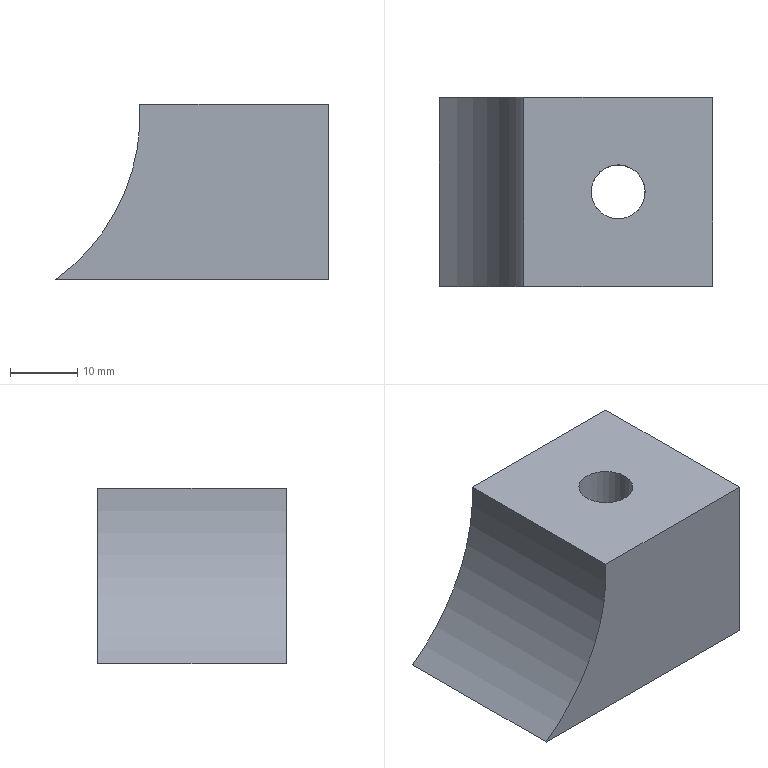Component | NX | SPACER_BLOCK | 1 solid | 7 faces | box 40.5 x 28 x 26 mm | volume 21611 mm3 | plane 5 | cylinder 2 | commonest cylinder face diameters 60 x1 8 x1
STEP:
#1=CARTESIAN_POINT('',(0.,0.,0.));
#2=DIRECTION('',(0.,0.,1.));
#3=DIRECTION('',(1.,0.,0.));
#4=AXIS2_PLACEMENT_3D('',#1,#2,#3);
#5=CARTESIAN_POINT('',(140.75,-66.75,19.));
#6=VERTEX_POINT('',#5);
#7=CARTESIAN_POINT('',(140.75,-70.75,19.));
#8=DIRECTION('',(0.,0.,1.));
#9=DIRECTION('',(0.,1.,0.));
#10=AXIS2_PLACEMENT_3D('',#7,#8,#9);
#11=CIRCLE('',#10,4.);
#12=CARTESIAN_POINT('',(154.75,-84.75,19.));
#13=DIRECTION('',(0.,0.,-1.));
#14=DIRECTION('',(0.,1.,0.));
#15=AXIS2_PLACEMENT_3D('',#12,#13,#14);
#16=PLANE('',#15);
#17=CARTESIAN_POINT('',(18.,-14.));
#18=CARTESIAN_POINT('',(18.,-20.928));
#19=CARTESIAN_POINT('',(12.,-17.464));
#20=CARTESIAN_POINT('',(6.,-14.));
#21=CARTESIAN_POINT('',(12.,-10.536));
#22=CARTESIAN_POINT('',(18.,-7.072));
#23=CARTESIAN_POINT('',(18.,-14.));
#24=(BOUNDED_CURVE()B_SPLINE_CURVE(2,(#17,#18,#19,#20,#21,#22,#23),.UNSPECIFIED.,.T.,.F.)B_SPLINE_CURVE_WITH_KNOTS((1,2,2,2,2,1),(-2.094,0.,2.094,4.189,6.283,8.378),.UNSPECIFIED.)CURVE()GEOMETRIC_REPRESENTATION_ITEM()RATIONAL_B_SPLINE_CURVE((1.,0.5,1.,0.5,1.,0.5,1.))REPRESENTATION_ITEM(''));
#25=(GEOMETRIC_REPRESENTATION_CONTEXT(2)PARAMETRIC_REPRESENTATION_CONTEXT()REPRESENTATION_CONTEXT('',''));
#26=DEFINITIONAL_REPRESENTATION('',(#24),#25);
#27=PCURVE('',#16,#26);
#28=CARTESIAN_POINT('',(140.75,-70.75,-5.));
#29=DIRECTION('',(-0.,0.,1.));
#30=DIRECTION('',(-1.,0.,-0.));
#31=AXIS2_PLACEMENT_3D('',#28,#29,#30);
#32=CYLINDRICAL_SURFACE('',#31,4.);
#33=CARTESIAN_POINT('',(4.712,24.));
#34=DIRECTION('',(1.,0.));
#35=VECTOR('',#34,1.);
#36=LINE('',#33,#35);
#37=(GEOMETRIC_REPRESENTATION_CONTEXT(2)PARAMETRIC_REPRESENTATION_CONTEXT()REPRESENTATION_CONTEXT('',''));
#38=DEFINITIONAL_REPRESENTATION('',(#36),#37);
#39=PCURVE('',#32,#38);
#40=SURFACE_CURVE('',#11,(#27,#39),.PCURVE_S1.);
#41=EDGE_CURVE('',#6,#6,#40,.T.);
#42=ORIENTED_EDGE('',*,*,#41,.T.);
#43=EDGE_LOOP('',(#42));
#44=FACE_BOUND('',#43,.T.);
#45=CARTESIAN_POINT('',(154.75,-56.75,19.));
#46=VERTEX_POINT('',#45);
#47=CARTESIAN_POINT('',(114.25,-56.75,19.));
#48=VERTEX_POINT('',#47);
#49=CARTESIAN_POINT('',(154.75,-56.75,19.));
#50=DIRECTION('',(-1.,0.,0.));
#51=VECTOR('',#50,1.);
#52=LINE('',#49,#51);
#53=CARTESIAN_POINT('',(28.,0.));
#54=DIRECTION('',(0.,-1.));
#55=VECTOR('',#54,1.);
#56=LINE('',#53,#55);
#57=(GEOMETRIC_REPRESENTATION_CONTEXT(2)PARAMETRIC_REPRESENTATION_CONTEXT()REPRESENTATION_CONTEXT('',''));
#58=DEFINITIONAL_REPRESENTATION('',(#56),#57);
#59=PCURVE('',#16,#58);
#60=CARTESIAN_POINT('',(96.793,-56.75,43.398));
#61=DIRECTION('',(0.,-1.,0.));
#62=DIRECTION('',(0.,0.,-1.));
#63=AXIS2_PLACEMENT_3D('',#60,#61,#62);
#64=PLANE('',#63);
#65=CARTESIAN_POINT('',(24.398,57.957));
#66=DIRECTION('',(0.,-1.));
#67=VECTOR('',#66,1.);
#68=LINE('',#65,#67);
#69=(GEOMETRIC_REPRESENTATION_CONTEXT(2)PARAMETRIC_REPRESENTATION_CONTEXT()REPRESENTATION_CONTEXT('',''));
#70=DEFINITIONAL_REPRESENTATION('',(#68),#69);
#71=PCURVE('',#64,#70);
#72=SURFACE_CURVE('',#52,(#59,#71),.PCURVE_S1.);
#73=EDGE_CURVE('',#46,#48,#72,.T.);
#74=ORIENTED_EDGE('',*,*,#73,.F.);
#75=CARTESIAN_POINT('',(154.75,-84.75,19.));
#76=VERTEX_POINT('',#75);
#77=CARTESIAN_POINT('',(154.75,-84.75,19.));
#78=DIRECTION('',(0.,1.,0.));
#79=VECTOR('',#78,1.);
#80=LINE('',#77,#79);
#81=CARTESIAN_POINT('',(0.,0.));
#82=DIRECTION('',(1.,0.));
#83=VECTOR('',#82,1.);
#84=LINE('',#81,#83);
#85=(GEOMETRIC_REPRESENTATION_CONTEXT(2)PARAMETRIC_REPRESENTATION_CONTEXT()REPRESENTATION_CONTEXT('',''));
#86=DEFINITIONAL_REPRESENTATION('',(#84),#85);
#87=PCURVE('',#16,#86);
#88=CARTESIAN_POINT('',(154.75,-84.75,45.));
#89=DIRECTION('',(1.,0.,0.));
#90=DIRECTION('',(0.,0.,1.));
#91=AXIS2_PLACEMENT_3D('',#88,#89,#90);
#92=PLANE('',#91);
#93=CARTESIAN_POINT('',(-26.,0.));
#94=DIRECTION('',(0.,-1.));
#95=VECTOR('',#94,1.);
#96=LINE('',#93,#95);
#97=(GEOMETRIC_REPRESENTATION_CONTEXT(2)PARAMETRIC_REPRESENTATION_CONTEXT()REPRESENTATION_CONTEXT('',''));
#98=DEFINITIONAL_REPRESENTATION('',(#96),#97);
#99=PCURVE('',#92,#98);
#100=SURFACE_CURVE('',#80,(#87,#99),.PCURVE_S1.);
#101=EDGE_CURVE('',#76,#46,#100,.T.);
#102=ORIENTED_EDGE('',*,*,#101,.F.);
#103=CARTESIAN_POINT('',(114.25,-84.75,19.));
#104=VERTEX_POINT('',#103);
#105=CARTESIAN_POINT('',(154.75,-84.75,19.));
#106=DIRECTION('',(-1.,0.,0.));
#107=VECTOR('',#106,1.);
#108=LINE('',#105,#107);
#109=CARTESIAN_POINT('',(0.,0.));
#110=DIRECTION('',(0.,-1.));
#111=VECTOR('',#110,1.);
#112=LINE('',#109,#111);
#113=(GEOMETRIC_REPRESENTATION_CONTEXT(2)PARAMETRIC_REPRESENTATION_CONTEXT()REPRESENTATION_CONTEXT('',''));
#114=DEFINITIONAL_REPRESENTATION('',(#112),#113);
#115=PCURVE('',#16,#114);
#116=CARTESIAN_POINT('',(96.793,-84.75,43.398));
#117=DIRECTION('',(0.,-1.,0.));
#118=DIRECTION('',(0.,0.,-1.));
#119=AXIS2_PLACEMENT_3D('',#116,#117,#118);
#120=PLANE('',#119);
#121=CARTESIAN_POINT('',(24.398,57.957));
#122=DIRECTION('',(0.,-1.));
#123=VECTOR('',#122,1.);
#124=LINE('',#121,#123);
#125=(GEOMETRIC_REPRESENTATION_CONTEXT(2)PARAMETRIC_REPRESENTATION_CONTEXT()REPRESENTATION_CONTEXT('',''));
#126=DEFINITIONAL_REPRESENTATION('',(#124),#125);
#127=PCURVE('',#120,#126);
#128=SURFACE_CURVE('',#108,(#115,#127),.PCURVE_S1.);
#129=EDGE_CURVE('',#76,#104,#128,.T.);
#130=ORIENTED_EDGE('',*,*,#129,.T.);
#131=CARTESIAN_POINT('',(114.25,-84.75,19.));
#132=DIRECTION('',(0.,1.,0.));
#133=VECTOR('',#132,1.);
#134=LINE('',#131,#133);
#135=CARTESIAN_POINT('',(0.,-40.5));
#136=DIRECTION('',(1.,0.));
#137=VECTOR('',#136,1.);
#138=LINE('',#135,#137);
#139=(GEOMETRIC_REPRESENTATION_CONTEXT(2)PARAMETRIC_REPRESENTATION_CONTEXT()REPRESENTATION_CONTEXT('',''));
#140=DEFINITIONAL_REPRESENTATION('',(#138),#139);
#141=PCURVE('',#16,#140);
#142=CARTESIAN_POINT('',(96.793,-84.75,43.398));
#143=DIRECTION('',(0.,1.,0.));
#144=DIRECTION('',(0.,0.,1.));
#145=AXIS2_PLACEMENT_3D('',#142,#143,#144);
#146=CYLINDRICAL_SURFACE('',#145,30.);
#147=CARTESIAN_POINT('',(2.521,0.));
#148=DIRECTION('',(0.,1.));
#149=VECTOR('',#148,1.);
#150=LINE('',#147,#149);
#151=(GEOMETRIC_REPRESENTATION_CONTEXT(2)PARAMETRIC_REPRESENTATION_CONTEXT()REPRESENTATION_CONTEXT('',''));
#152=DEFINITIONAL_REPRESENTATION('',(#150),#151);
#153=PCURVE('',#146,#152);
#154=SURFACE_CURVE('',#134,(#141,#153),.PCURVE_S1.);
#155=EDGE_CURVE('',#104,#48,#154,.T.);
#156=ORIENTED_EDGE('',*,*,#155,.T.);
#157=EDGE_LOOP('',(#74,#102,#130,#156));
#158=FACE_BOUND('',#157,.T.);
#159=ADVANCED_FACE('',(#44,#158),#16,.T.);
#160=CARTESIAN_POINT('',(126.75,-84.75,45.));
#161=VERTEX_POINT('',#160);
#162=CARTESIAN_POINT('',(126.75,-56.75,45.));
#163=VERTEX_POINT('',#162);
#164=CARTESIAN_POINT('',(126.75,-84.75,45.));
#165=DIRECTION('',(0.,1.,0.));
#166=VECTOR('',#165,1.);
#167=LINE('',#164,#166);
#168=CARTESIAN_POINT('',(1.517,0.));
#169=DIRECTION('',(0.,1.));
#170=VECTOR('',#169,1.);
#171=LINE('',#168,#170);
#172=(GEOMETRIC_REPRESENTATION_CONTEXT(2)PARAMETRIC_REPRESENTATION_CONTEXT()REPRESENTATION_CONTEXT('',''));
#173=DEFINITIONAL_REPRESENTATION('',(#171),#172);
#174=PCURVE('',#146,#173);
#175=CARTESIAN_POINT('',(126.75,-84.75,45.));
#176=DIRECTION('',(-0.,0.,1.));
#177=DIRECTION('',(-1.,0.,-0.));
#178=AXIS2_PLACEMENT_3D('',#175,#176,#177);
#179=PLANE('',#178);
#180=CARTESIAN_POINT('',(0.,0.));
#181=DIRECTION('',(0.,-1.));
#182=VECTOR('',#181,1.);
#183=LINE('',#180,#182);
#184=(GEOMETRIC_REPRESENTATION_CONTEXT(2)PARAMETRIC_REPRESENTATION_CONTEXT()REPRESENTATION_CONTEXT('',''));
#185=DEFINITIONAL_REPRESENTATION('',(#183),#184);
#186=PCURVE('',#179,#185);
#187=SURFACE_CURVE('',#167,(#174,#186),.PCURVE_S1.);
#188=EDGE_CURVE('',#161,#163,#187,.T.);
#189=ORIENTED_EDGE('',*,*,#188,.F.);
#190=CARTESIAN_POINT('',(96.793,-84.75,43.398));
#191=DIRECTION('',(0.,-1.,0.));
#192=DIRECTION('',(1.,0.,0.));
#193=AXIS2_PLACEMENT_3D('',#190,#191,#192);
#194=CIRCLE('',#193,30.);
#195=CARTESIAN_POINT('',(7.854,0.));
#196=DIRECTION('',(-1.,0.));
#197=VECTOR('',#196,1.);
#198=LINE('',#195,#197);
#199=(GEOMETRIC_REPRESENTATION_CONTEXT(2)PARAMETRIC_REPRESENTATION_CONTEXT()REPRESENTATION_CONTEXT('',''));
#200=DEFINITIONAL_REPRESENTATION('',(#198),#199);
#201=PCURVE('',#146,#200);
#202=CARTESIAN_POINT('',(0.,0.));
#203=DIRECTION('',(0.,1.));
#204=AXIS2_PLACEMENT_2D('',#202,#203);
#205=CIRCLE('',#204,30.);
#206=(GEOMETRIC_REPRESENTATION_CONTEXT(2)PARAMETRIC_REPRESENTATION_CONTEXT()REPRESENTATION_CONTEXT('',''));
#207=DEFINITIONAL_REPRESENTATION('',(#205),#206);
#208=PCURVE('',#120,#207);
#209=SURFACE_CURVE('',#194,(#201,#208),.PCURVE_S1.);
#210=EDGE_CURVE('',#104,#161,#209,.T.);
#211=ORIENTED_EDGE('',*,*,#210,.F.);
#212=ORIENTED_EDGE('',*,*,#155,.T.);
#213=CARTESIAN_POINT('',(96.793,-56.75,43.398));
#214=DIRECTION('',(0.,-1.,0.));
#215=DIRECTION('',(1.,0.,0.));
#216=AXIS2_PLACEMENT_3D('',#213,#214,#215);
#217=CIRCLE('',#216,30.);
#218=CARTESIAN_POINT('',(7.854,28.));
#219=DIRECTION('',(-1.,0.));
#220=VECTOR('',#219,1.);
#221=LINE('',#218,#220);
#222=(GEOMETRIC_REPRESENTATION_CONTEXT(2)PARAMETRIC_REPRESENTATION_CONTEXT()REPRESENTATION_CONTEXT('',''));
#223=DEFINITIONAL_REPRESENTATION('',(#221),#222);
#224=PCURVE('',#146,#223);
#225=CARTESIAN_POINT('',(0.,0.));
#226=DIRECTION('',(0.,1.));
#227=AXIS2_PLACEMENT_2D('',#225,#226);
#228=CIRCLE('',#227,30.);
#229=(GEOMETRIC_REPRESENTATION_CONTEXT(2)PARAMETRIC_REPRESENTATION_CONTEXT()REPRESENTATION_CONTEXT('',''));
#230=DEFINITIONAL_REPRESENTATION('',(#228),#229);
#231=PCURVE('',#64,#230);
#232=SURFACE_CURVE('',#217,(#224,#231),.PCURVE_S1.);
#233=EDGE_CURVE('',#48,#163,#232,.T.);
#234=ORIENTED_EDGE('',*,*,#233,.T.);
#235=EDGE_LOOP('',(#189,#211,#212,#234));
#236=FACE_BOUND('',#235,.F.);
#237=ADVANCED_FACE('',(#236),#146,.F.);
#238=CARTESIAN_POINT('',(144.75,-70.75,45.));
#239=VERTEX_POINT('',#238);
#240=CARTESIAN_POINT('',(140.75,-66.75,45.));
#241=VERTEX_POINT('',#240);
#242=CARTESIAN_POINT('',(140.75,-70.75,45.));
#243=DIRECTION('',(0.,0.,-1.));
#244=DIRECTION('',(1.,0.,0.));
#245=AXIS2_PLACEMENT_3D('',#242,#243,#244);
#246=CIRCLE('',#245,4.);
#247=CARTESIAN_POINT('',(-18.,-14.));
#248=CARTESIAN_POINT('',(-18.,-7.072));
#249=CARTESIAN_POINT('',(-12.,-10.536));
#250=CARTESIAN_POINT('',(-6.,-14.));
#251=CARTESIAN_POINT('',(-12.,-17.464));
#252=CARTESIAN_POINT('',(-18.,-20.928));
#253=CARTESIAN_POINT('',(-18.,-14.));
#254=(BOUNDED_CURVE()B_SPLINE_CURVE(2,(#247,#248,#249,#250,#251,#252,#253),.UNSPECIFIED.,.T.,.F.)B_SPLINE_CURVE_WITH_KNOTS((1,2,2,2,2,1),(-2.094,0.,2.094,4.189,6.283,8.378),.UNSPECIFIED.)CURVE()GEOMETRIC_REPRESENTATION_ITEM()RATIONAL_B_SPLINE_CURVE((1.,0.5,1.,0.5,1.,0.5,1.))REPRESENTATION_ITEM(''));
#255=(GEOMETRIC_REPRESENTATION_CONTEXT(2)PARAMETRIC_REPRESENTATION_CONTEXT()REPRESENTATION_CONTEXT('',''));
#256=DEFINITIONAL_REPRESENTATION('',(#254),#255);
#257=PCURVE('',#179,#256);
#258=CARTESIAN_POINT('',(9.425,50.));
#259=DIRECTION('',(-1.,0.));
#260=VECTOR('',#259,1.);
#261=LINE('',#258,#260);
#262=(GEOMETRIC_REPRESENTATION_CONTEXT(2)PARAMETRIC_REPRESENTATION_CONTEXT()REPRESENTATION_CONTEXT('',''));
#263=DEFINITIONAL_REPRESENTATION('',(#261),#262);
#264=PCURVE('',#32,#263);
#265=SURFACE_CURVE('',#246,(#257,#264),.PCURVE_S1.);
#266=EDGE_CURVE('',#239,#241,#265,.T.);
#267=ORIENTED_EDGE('',*,*,#266,.T.);
#268=CARTESIAN_POINT('',(140.75,-70.75,45.));
#269=DIRECTION('',(0.,0.,-1.));
#270=DIRECTION('',(1.,0.,0.));
#271=AXIS2_PLACEMENT_3D('',#268,#269,#270);
#272=CIRCLE('',#271,4.);
#273=CARTESIAN_POINT('',(-18.,-14.));
#274=CARTESIAN_POINT('',(-18.,-7.072));
#275=CARTESIAN_POINT('',(-12.,-10.536));
#276=CARTESIAN_POINT('',(-6.,-14.));
#277=CARTESIAN_POINT('',(-12.,-17.464));
#278=CARTESIAN_POINT('',(-18.,-20.928));
#279=CARTESIAN_POINT('',(-18.,-14.));
#280=(BOUNDED_CURVE()B_SPLINE_CURVE(2,(#273,#274,#275,#276,#277,#278,#279),.UNSPECIFIED.,.T.,.F.)B_SPLINE_CURVE_WITH_KNOTS((1,2,2,2,2,1),(-2.094,0.,2.094,4.189,6.283,8.378),.UNSPECIFIED.)CURVE()GEOMETRIC_REPRESENTATION_ITEM()RATIONAL_B_SPLINE_CURVE((1.,0.5,1.,0.5,1.,0.5,1.))REPRESENTATION_ITEM(''));
#281=(GEOMETRIC_REPRESENTATION_CONTEXT(2)PARAMETRIC_REPRESENTATION_CONTEXT()REPRESENTATION_CONTEXT('',''));
#282=DEFINITIONAL_REPRESENTATION('',(#280),#281);
#283=PCURVE('',#179,#282);
#284=CARTESIAN_POINT('',(15.708,50.));
#285=DIRECTION('',(-1.,0.));
#286=VECTOR('',#285,1.);
#287=LINE('',#284,#286);
#288=(GEOMETRIC_REPRESENTATION_CONTEXT(2)PARAMETRIC_REPRESENTATION_CONTEXT()REPRESENTATION_CONTEXT('',''));
#289=DEFINITIONAL_REPRESENTATION('',(#287),#288);
#290=PCURVE('',#32,#289);
#291=SURFACE_CURVE('',#272,(#283,#290),.PCURVE_S1.);
#292=EDGE_CURVE('',#241,#239,#291,.T.);
#293=ORIENTED_EDGE('',*,*,#292,.T.);
#294=EDGE_LOOP('',(#267,#293));
#295=FACE_BOUND('',#294,.T.);
#296=CARTESIAN_POINT('',(154.75,-56.75,45.));
#297=VERTEX_POINT('',#296);
#298=CARTESIAN_POINT('',(126.75,-56.75,45.));
#299=DIRECTION('',(1.,0.,0.));
#300=VECTOR('',#299,1.);
#301=LINE('',#298,#300);
#302=CARTESIAN_POINT('',(0.,-28.));
#303=DIRECTION('',(-1.,0.));
#304=VECTOR('',#303,1.);
#305=LINE('',#302,#304);
#306=(GEOMETRIC_REPRESENTATION_CONTEXT(2)PARAMETRIC_REPRESENTATION_CONTEXT()REPRESENTATION_CONTEXT('',''));
#307=DEFINITIONAL_REPRESENTATION('',(#305),#306);
#308=PCURVE('',#179,#307);
#309=CARTESIAN_POINT('',(-1.602,29.957));
#310=DIRECTION('',(-0.,1.));
#311=VECTOR('',#310,1.);
#312=LINE('',#309,#311);
#313=(GEOMETRIC_REPRESENTATION_CONTEXT(2)PARAMETRIC_REPRESENTATION_CONTEXT()REPRESENTATION_CONTEXT('',''));
#314=DEFINITIONAL_REPRESENTATION('',(#312),#313);
#315=PCURVE('',#64,#314);
#316=SURFACE_CURVE('',#301,(#308,#315),.PCURVE_S1.);
#317=EDGE_CURVE('',#163,#297,#316,.T.);
#318=ORIENTED_EDGE('',*,*,#317,.F.);
#319=ORIENTED_EDGE('',*,*,#188,.F.);
#320=CARTESIAN_POINT('',(154.75,-84.75,45.));
#321=VERTEX_POINT('',#320);
#322=CARTESIAN_POINT('',(126.75,-84.75,45.));
#323=DIRECTION('',(1.,0.,0.));
#324=VECTOR('',#323,1.);
#325=LINE('',#322,#324);
#326=CARTESIAN_POINT('',(0.,0.));
#327=DIRECTION('',(-1.,0.));
#328=VECTOR('',#327,1.);
#329=LINE('',#326,#328);
#330=(GEOMETRIC_REPRESENTATION_CONTEXT(2)PARAMETRIC_REPRESENTATION_CONTEXT()REPRESENTATION_CONTEXT('',''));
#331=DEFINITIONAL_REPRESENTATION('',(#329),#330);
#332=PCURVE('',#179,#331);
#333=CARTESIAN_POINT('',(-1.602,29.957));
#334=DIRECTION('',(-0.,1.));
#335=VECTOR('',#334,1.);
#336=LINE('',#333,#335);
#337=(GEOMETRIC_REPRESENTATION_CONTEXT(2)PARAMETRIC_REPRESENTATION_CONTEXT()REPRESENTATION_CONTEXT('',''));
#338=DEFINITIONAL_REPRESENTATION('',(#336),#337);
#339=PCURVE('',#120,#338);
#340=SURFACE_CURVE('',#325,(#332,#339),.PCURVE_S1.);
#341=EDGE_CURVE('',#161,#321,#340,.T.);
#342=ORIENTED_EDGE('',*,*,#341,.T.);
#343=CARTESIAN_POINT('',(154.75,-84.75,45.));
#344=DIRECTION('',(0.,1.,0.));
#345=VECTOR('',#344,1.);
#346=LINE('',#343,#345);
#347=CARTESIAN_POINT('',(-28.,0.));
#348=DIRECTION('',(0.,-1.));
#349=VECTOR('',#348,1.);
#350=LINE('',#347,#349);
#351=(GEOMETRIC_REPRESENTATION_CONTEXT(2)PARAMETRIC_REPRESENTATION_CONTEXT()REPRESENTATION_CONTEXT('',''));
#352=DEFINITIONAL_REPRESENTATION('',(#350),#351);
#353=PCURVE('',#179,#352);
#354=CARTESIAN_POINT('',(0.,0.));
#355=DIRECTION('',(0.,-1.));
#356=VECTOR('',#355,1.);
#357=LINE('',#354,#356);
#358=(GEOMETRIC_REPRESENTATION_CONTEXT(2)PARAMETRIC_REPRESENTATION_CONTEXT()REPRESENTATION_CONTEXT('',''));
#359=DEFINITIONAL_REPRESENTATION('',(#357),#358);
#360=PCURVE('',#92,#359);
#361=SURFACE_CURVE('',#346,(#353,#360),.PCURVE_S1.);
#362=EDGE_CURVE('',#321,#297,#361,.T.);
#363=ORIENTED_EDGE('',*,*,#362,.T.);
#364=EDGE_LOOP('',(#318,#319,#342,#363));
#365=FACE_BOUND('',#364,.T.);
#366=ADVANCED_FACE('',(#295,#365),#179,.T.);
#367=CARTESIAN_POINT('',(154.75,-56.75,45.));
#368=DIRECTION('',(0.,0.,-1.));
#369=VECTOR('',#368,1.);
#370=LINE('',#367,#369);
#371=CARTESIAN_POINT('',(0.,-28.));
#372=DIRECTION('',(-1.,0.));
#373=VECTOR('',#372,1.);
#374=LINE('',#371,#373);
#375=(GEOMETRIC_REPRESENTATION_CONTEXT(2)PARAMETRIC_REPRESENTATION_CONTEXT()REPRESENTATION_CONTEXT('',''));
#376=DEFINITIONAL_REPRESENTATION('',(#374),#375);
#377=PCURVE('',#92,#376);
#378=CARTESIAN_POINT('',(-1.602,57.957));
#379=DIRECTION('',(1.,0.));
#380=VECTOR('',#379,1.);
#381=LINE('',#378,#380);
#382=(GEOMETRIC_REPRESENTATION_CONTEXT(2)PARAMETRIC_REPRESENTATION_CONTEXT()REPRESENTATION_CONTEXT('',''));
#383=DEFINITIONAL_REPRESENTATION('',(#381),#382);
#384=PCURVE('',#64,#383);
#385=SURFACE_CURVE('',#370,(#377,#384),.PCURVE_S1.);
#386=EDGE_CURVE('',#297,#46,#385,.T.);
#387=ORIENTED_EDGE('',*,*,#386,.F.);
#388=ORIENTED_EDGE('',*,*,#362,.F.);
#389=CARTESIAN_POINT('',(154.75,-84.75,45.));
#390=DIRECTION('',(0.,0.,-1.));
#391=VECTOR('',#390,1.);
#392=LINE('',#389,#391);
#393=CARTESIAN_POINT('',(0.,0.));
#394=DIRECTION('',(-1.,0.));
#395=VECTOR('',#394,1.);
#396=LINE('',#393,#395);
#397=(GEOMETRIC_REPRESENTATION_CONTEXT(2)PARAMETRIC_REPRESENTATION_CONTEXT()REPRESENTATION_CONTEXT('',''));
#398=DEFINITIONAL_REPRESENTATION('',(#396),#397);
#399=PCURVE('',#92,#398);
#400=CARTESIAN_POINT('',(-1.602,57.957));
#401=DIRECTION('',(1.,0.));
#402=VECTOR('',#401,1.);
#403=LINE('',#400,#402);
#404=(GEOMETRIC_REPRESENTATION_CONTEXT(2)PARAMETRIC_REPRESENTATION_CONTEXT()REPRESENTATION_CONTEXT('',''));
#405=DEFINITIONAL_REPRESENTATION('',(#403),#404);
#406=PCURVE('',#120,#405);
#407=SURFACE_CURVE('',#392,(#399,#406),.PCURVE_S1.);
#408=EDGE_CURVE('',#321,#76,#407,.T.);
#409=ORIENTED_EDGE('',*,*,#408,.T.);
#410=ORIENTED_EDGE('',*,*,#101,.T.);
#411=EDGE_LOOP('',(#387,#388,#409,#410));
#412=FACE_BOUND('',#411,.T.);
#413=ADVANCED_FACE('',(#412),#92,.T.);
#414=ORIENTED_EDGE('',*,*,#129,.F.);
#415=ORIENTED_EDGE('',*,*,#408,.F.);
#416=ORIENTED_EDGE('',*,*,#341,.F.);
#417=ORIENTED_EDGE('',*,*,#210,.F.);
#418=EDGE_LOOP('',(#414,#415,#416,#417));
#419=FACE_BOUND('',#418,.T.);
#420=ADVANCED_FACE('',(#419),#120,.T.);
#421=ORIENTED_EDGE('',*,*,#73,.T.);
#422=ORIENTED_EDGE('',*,*,#233,.T.);
#423=ORIENTED_EDGE('',*,*,#317,.T.);
#424=ORIENTED_EDGE('',*,*,#386,.T.);
#425=EDGE_LOOP('',(#421,#422,#423,#424));
#426=FACE_BOUND('',#425,.T.);
#427=ADVANCED_FACE('',(#426),#64,.F.);
#428=ORIENTED_EDGE('',*,*,#41,.T.);
#429=CARTESIAN_POINT('',(140.75,-66.75,19.));
#430=CARTESIAN_POINT('',(140.75,-66.75,45.));
#431=B_SPLINE_CURVE_WITH_KNOTS('',1,(#429,#430),.UNSPECIFIED.,.F.,.F.,(2,2),(24.,50.),.PIECEWISE_BEZIER_KNOTS.);
#432=CARTESIAN_POINT('',(10.996,0.));
#433=DIRECTION('',(0.,1.));
#434=VECTOR('',#433,1.);
#435=LINE('',#432,#434);
#436=(GEOMETRIC_REPRESENTATION_CONTEXT(2)PARAMETRIC_REPRESENTATION_CONTEXT()REPRESENTATION_CONTEXT('',''));
#437=DEFINITIONAL_REPRESENTATION('',(#435),#436);
#438=PCURVE('',#32,#437);
#439=CARTESIAN_POINT('',(4.712,0.));
#440=DIRECTION('',(0.,1.));
#441=VECTOR('',#440,1.);
#442=LINE('',#439,#441);
#443=(GEOMETRIC_REPRESENTATION_CONTEXT(2)PARAMETRIC_REPRESENTATION_CONTEXT()REPRESENTATION_CONTEXT('',''));
#444=DEFINITIONAL_REPRESENTATION('',(#442),#443);
#445=PCURVE('',#32,#444);
#446=SEAM_CURVE('',#431,(#438,#445),.PCURVE_S1.);
#447=EDGE_CURVE('',#6,#241,#446,.T.);
#448=ORIENTED_EDGE('',*,*,#447,.T.);
#449=ORIENTED_EDGE('',*,*,#292,.T.);
#450=ORIENTED_EDGE('',*,*,#266,.T.);
#451=ORIENTED_EDGE('',*,*,#447,.F.);
#452=EDGE_LOOP('',(#428,#448,#449,#450,#451));
#453=FACE_BOUND('',#452,.F.);
#454=ADVANCED_FACE('',(#453),#32,.F.);
#455=CLOSED_SHELL('',(#159,#237,#366,#413,#420,#427,#454));
#456=MANIFOLD_SOLID_BREP('',#455);
#457=(LENGTH_UNIT()NAMED_UNIT(*)SI_UNIT(.MILLI.,.METRE.));
#458=UNCERTAINTY_MEASURE_WITH_UNIT(LENGTH_MEASURE(0.000002),#457,'','');
#459=(NAMED_UNIT(*)PLANE_ANGLE_UNIT()SI_UNIT($,.RADIAN.));
#460=(NAMED_UNIT(*)SI_UNIT($,.STERADIAN.)SOLID_ANGLE_UNIT());
#461=(GEOMETRIC_REPRESENTATION_CONTEXT(3)GLOBAL_UNCERTAINTY_ASSIGNED_CONTEXT((#458))GLOBAL_UNIT_ASSIGNED_CONTEXT((#457,#459,#460))REPRESENTATION_CONTEXT('',''));
#462=ADVANCED_BREP_SHAPE_REPRESENTATION('',(#4,#456),#461);